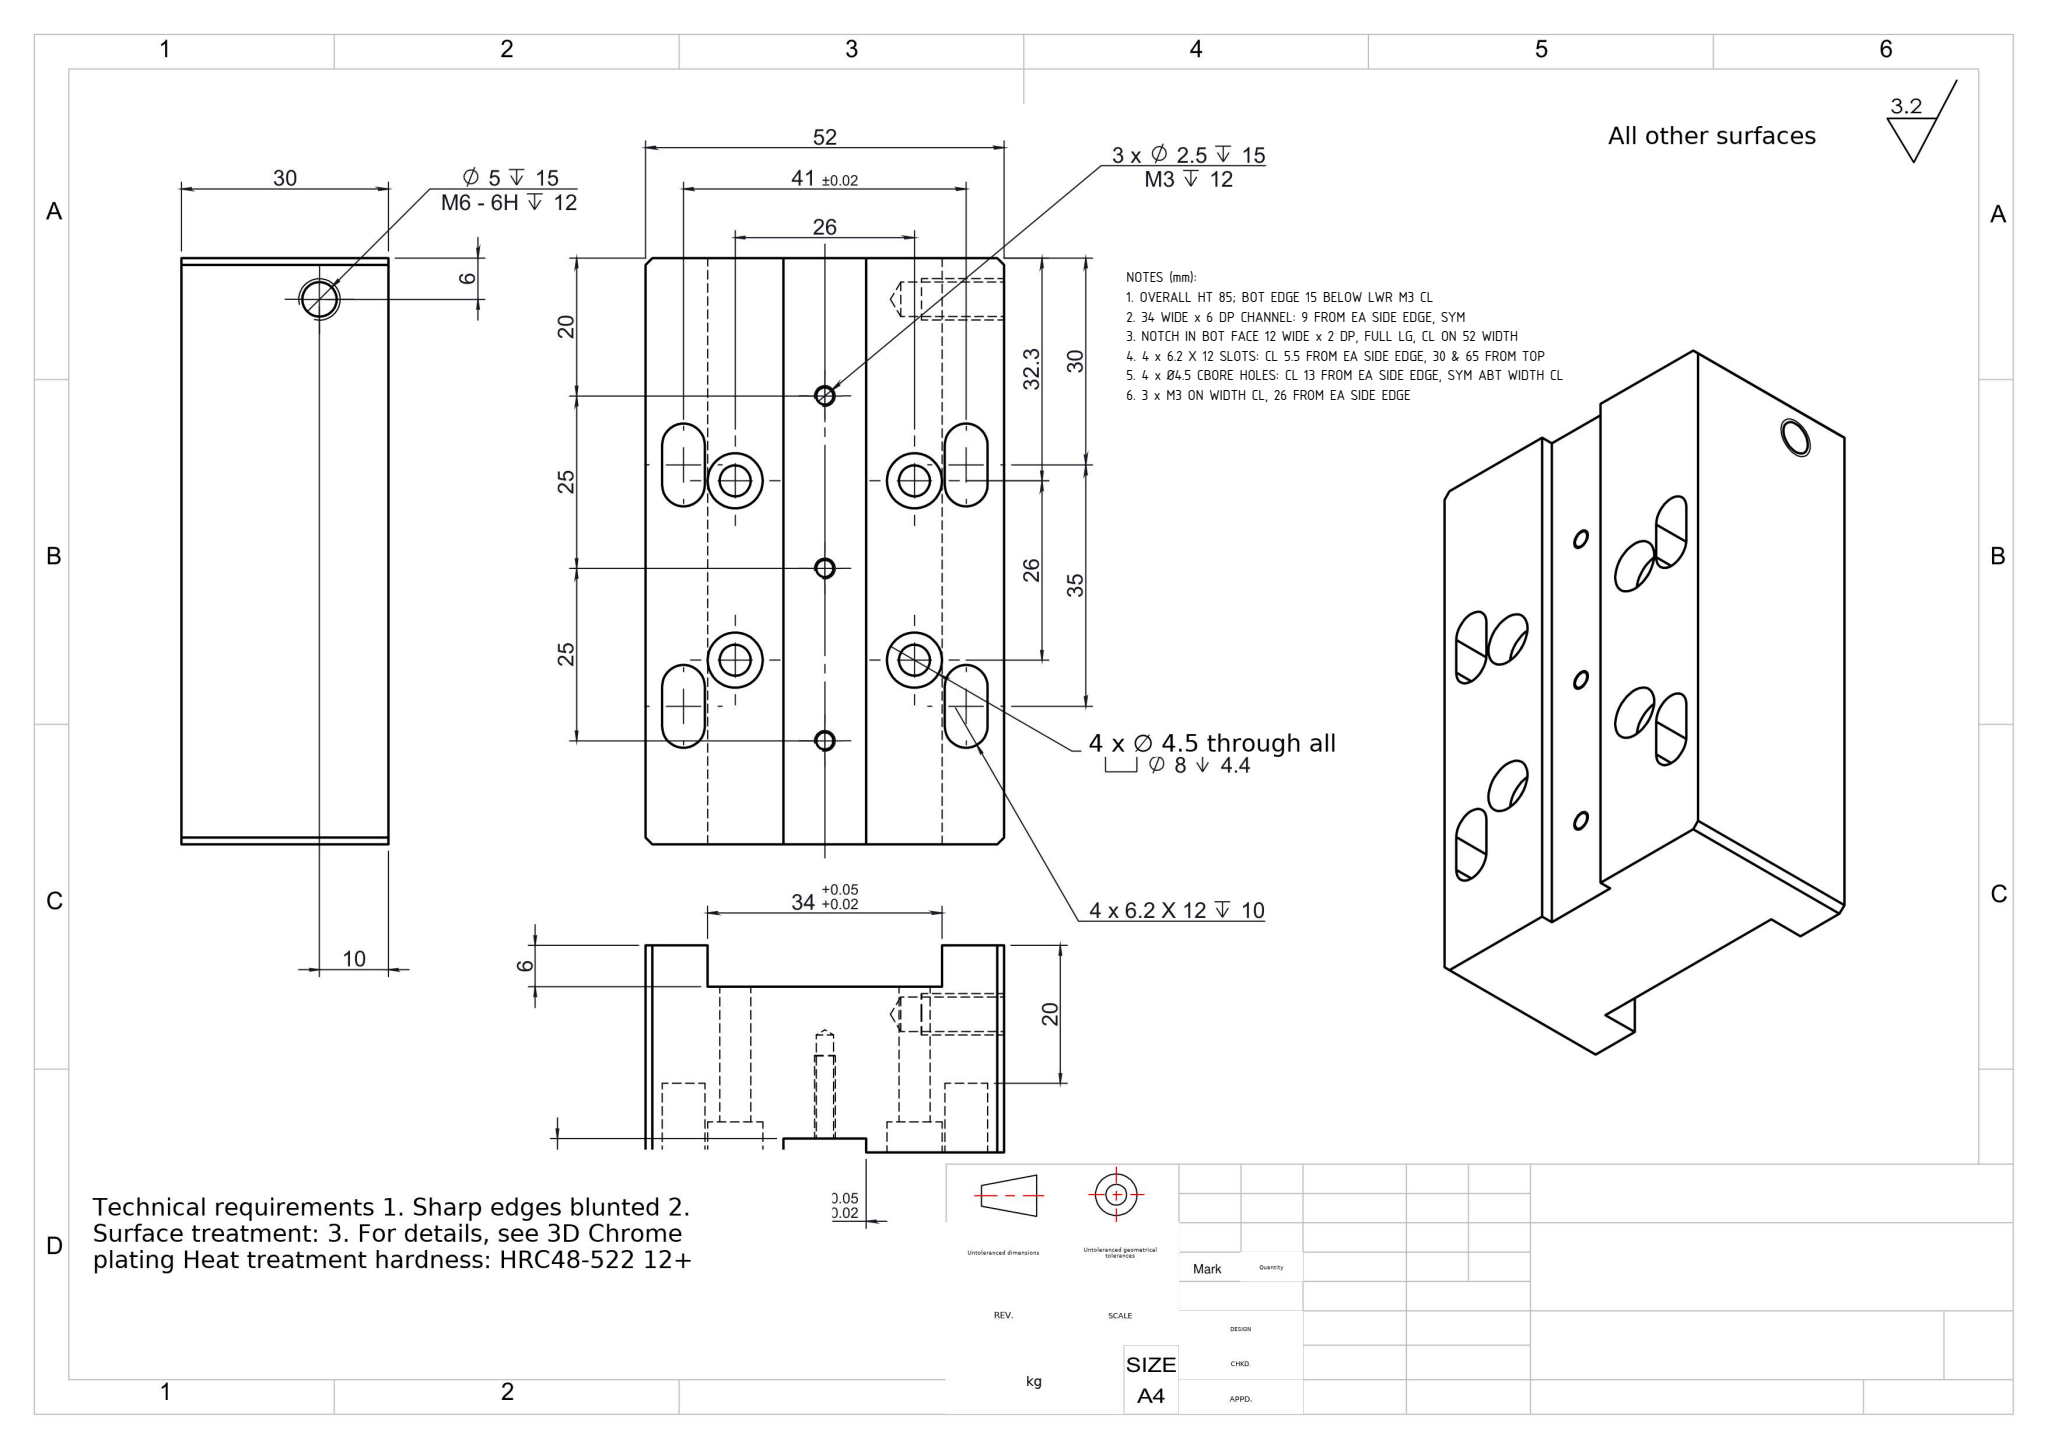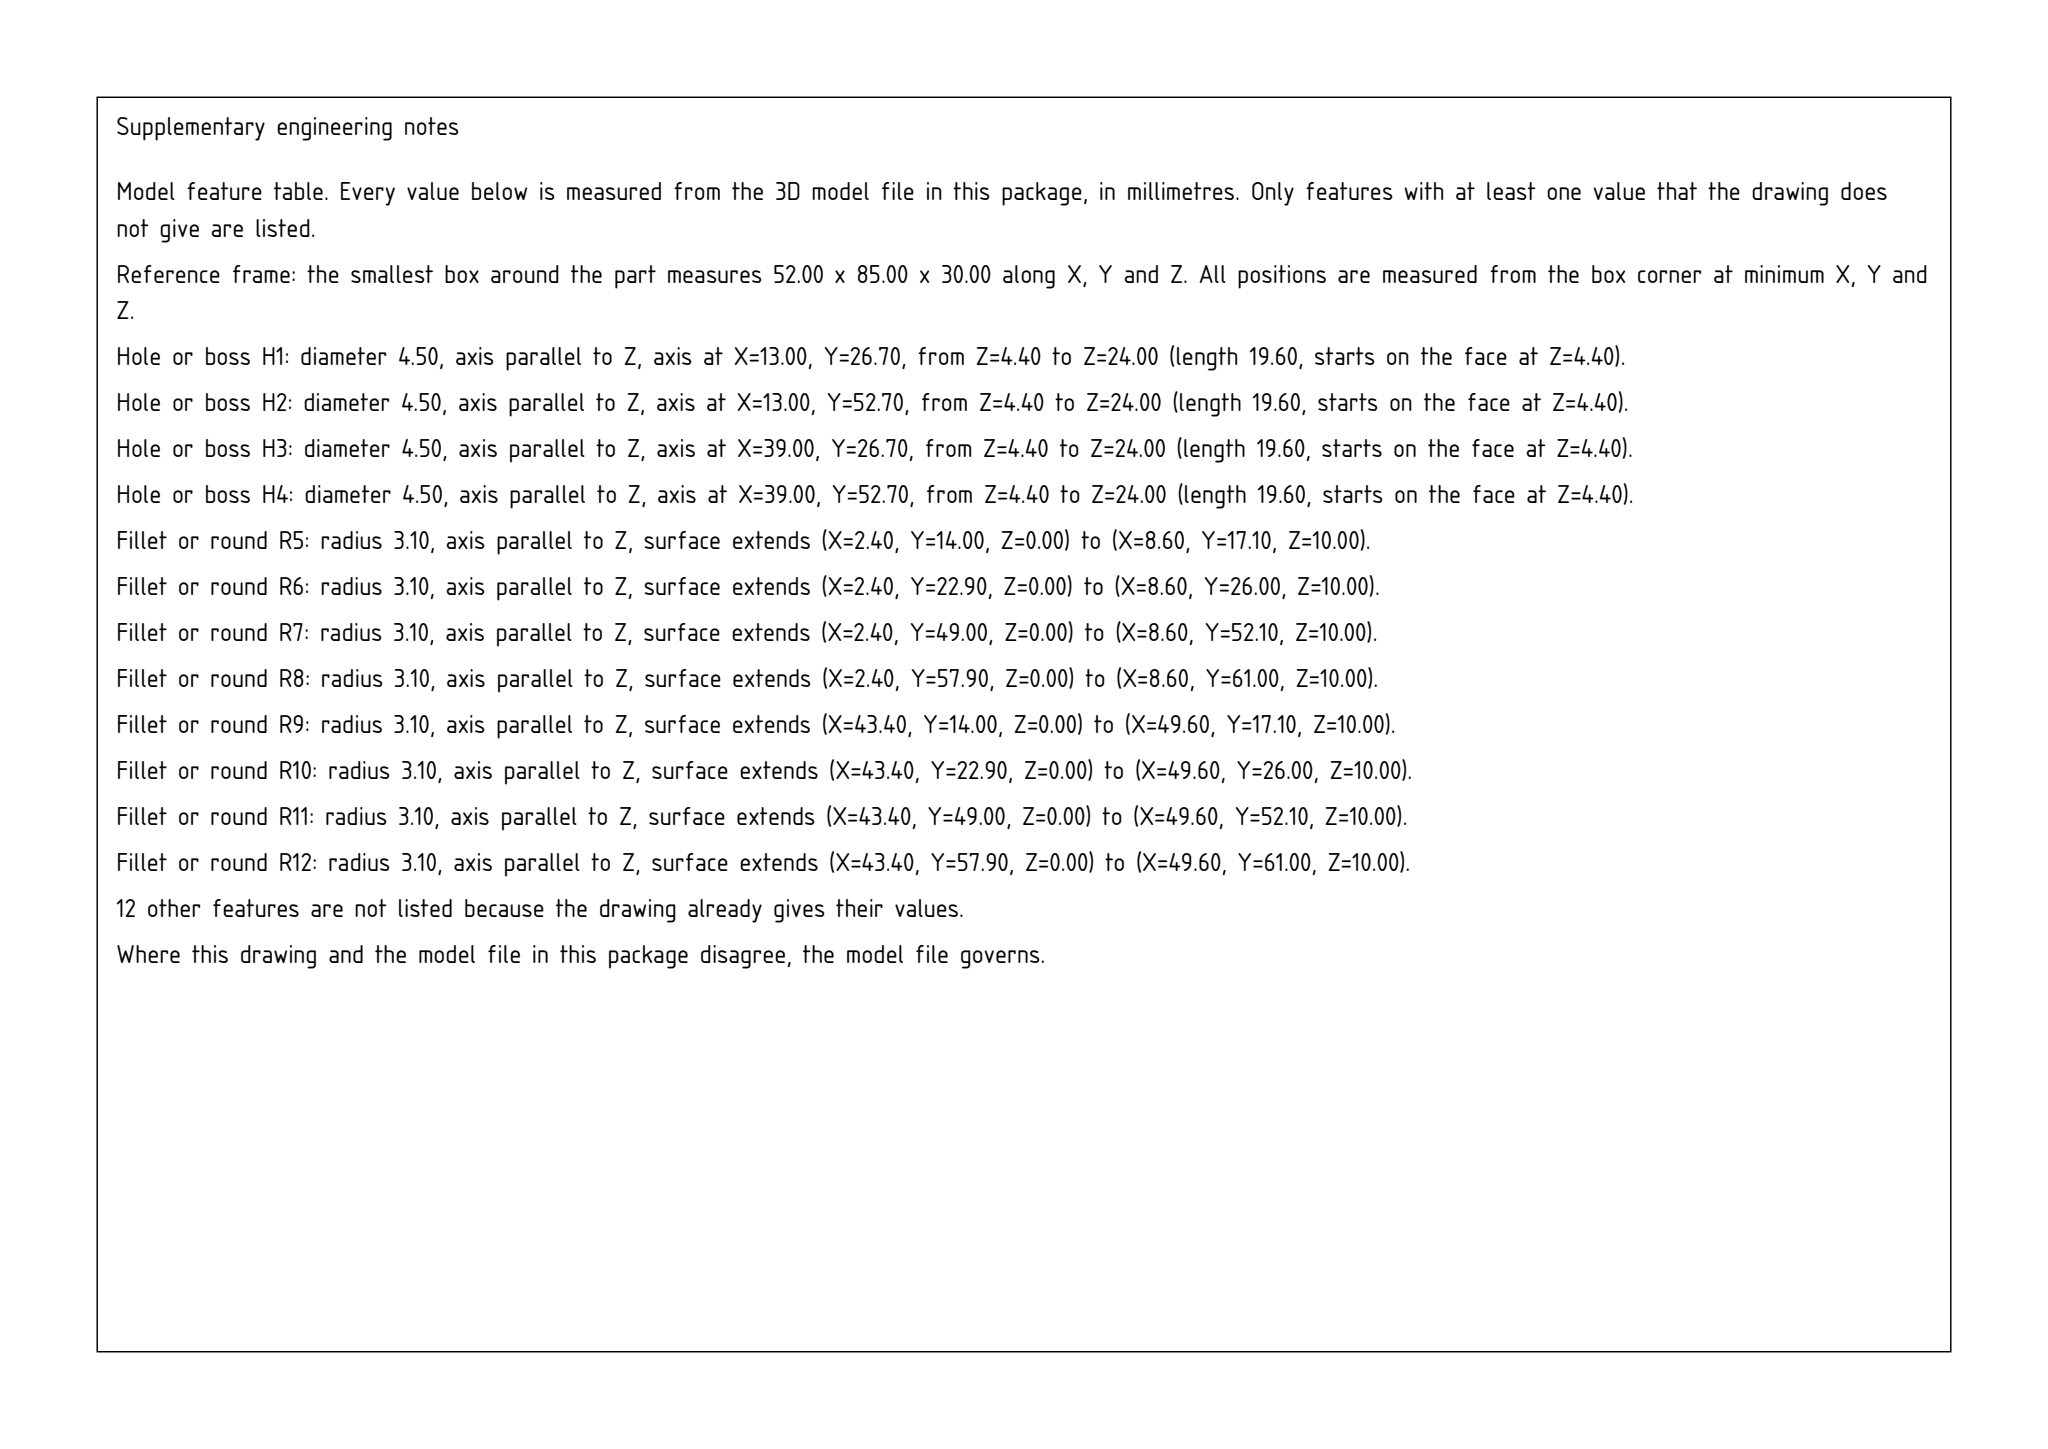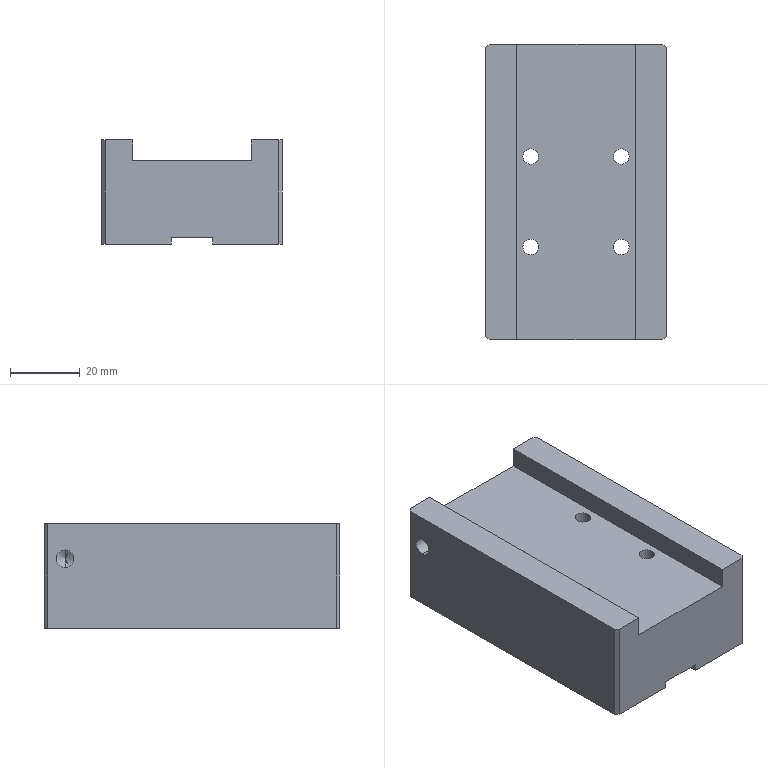Part | SolidWorks | mm | 1 solid | 74 faces | box 52 x 85 x 30 mm | volume 107853 mm3 | plane 34 | cylinder 32 | cone 8 | commonest cylinder face diameters 8 x8 4.5 x8 6.2 x8 2.5 x6 5 x2
Drawing notes:
OVERALL HT 85; BOT EDGE 15 BELOW LWR M3 CL | from the solid: bbox Y=85; M3 at y=15,40,65 -> 20+25+25+15=85
34 WIDE x 6 DP CHANNEL: 9 FROM EA SIDE EDGE, SYM | from the solid: x-planes 9.0 & 43.0 in 52 width; z 24.0-30.0 = 6 DP
NOTCH IN BOT FACE 12 WIDE x 2 DP, FULL LG, CL ON 52 WIDTH | from the solid: x planes 20 & 32 (12 wide, CL 26); notch floor z=2
4 x 6.2 X 12 SLOTS: CL 5.5 FROM EA SIDE EDGE, 30 & 65 FROM TOP | from the solid: Ø6.2 ends x=5.5 & 46.5; y 17.1/22.9 & 52.1/57.9 -> CL 20 & 55 from btm
4 x Ø4.5 CBORE HOLES: CL 13 FROM EA SIDE EDGE, SYM ABT WIDTH CL | from the solid: Ø4.5/Ø8 at x=13 & 39 of 52 wide; spacing 26
3 x M3 ON WIDTH CL, 26 FROM EA SIDE EDGE | from the solid: Ø2.5 holes at x=26.0 in 52 wide bbox